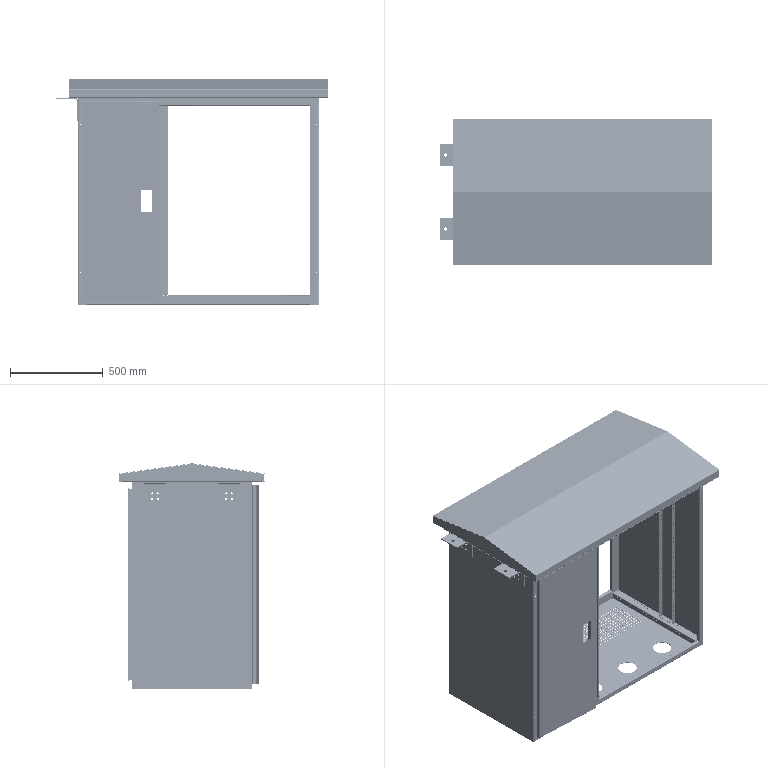Assembly | SolidWorks | mm | 23 component files | 23 solids | 4118 faces | box 1470 x 790 x 1217.97 mm | volume 9952438 mm3 | cylinder 2496 | plane 1582 | spline 40 | commonest cylinder face diameters 5 x1062 7 x724 5.4 x416 6 x80 3 x68 9 x40 13 x32 4 x20
Bill of materials:
BottomPlate4 | 1 |  | Rectangular sheet-metal tray-like panel: flat base with upturned walls along both long edges, each ending in a short outward flange, perforated by large round holes and arrays of short slots.
BottomPlateMiddleBeam | 1 |  | Long straight U-channel (open three-sided section, rounded bends) perforated with regularly spaced round holes on the web and both legs.
BottomSideBeam | 2 |  | Long straight channel with an asymmetric profile: web with one short leg and one long leg ending in an inward return lip; single rows of round holes on two faces.
BoxSidePlate01 | 2 |  | Flat rectangular sheet panel with formed flanges along two opposite edges, two clusters of four small holes near one end, and small holes in the flanges.
BoxUpperBeam2 | 1 |  | Long formed sheet-metal rail with a stepped Z/J-like profile (top flange, tall web, bottom flange, short upturned lip), with a row of oblong holes in the top flange and a rectangular notch in the lower flange.
BoxUpperBeam2Rear | 1 |  | Long formed sheet-metal rail with a stepped profile like the previous rail but mirrored, with four holes along one flange and a rectangular notch.
DoorPanel415 | 1 |  | Flat rectangular plate with a single off-center rectangular through-cutout.
LiftingBentPlate | 2 |  | Sheet-metal L-shaped angle bracket with a generous bend radius; one leg has one larger round hole, the other leg has a 2x2 pattern of four smaller round holes.
MiddleColumn3 | 2 |  | Long straight lipped C-channel with rounded corners and inward-turned lips, with no visible holes.
MountingColumn | 2 |  | Tall slender closed or folded rectangular-section post with a single row of small round holes along one narrow face and an end face with two oblong slots.
MountingColumnMiddle | 1 |  | Tall rectangular-section post, wider than the similar single-row post, with two rows of small round holes along one face and an end face with four oblong slots in a 2x2 pattern.
TopCover | 1 |  | Rectangular sheet-metal cover with a shallow peaked (gabled) top: two sloped panels meet at a central ridge, with short downturned side flanges ending in small inward lips.
TopCoverEndPlate | 2 |  | Thin flat sheet panel with a five-sided outline: a rectangle with a shallow triangular peak along one long edge. A narrow flange is bent at 90 degrees along the opposite straight long edge, with a small inside bend radius, so the cross-section is L-shaped.
TopCoverFrontAndRearFlange | 2 |  | Long, narrow sheet-metal strip with a Z-shaped (joggle) offset cross-section that forms two parallel flat flanges at different levels. The wider flange has one long row of many evenly spaced, identical narrow slots running along its length. The other flange is a little shorter, which leaves a step at each end, and has four small round or slightly oblong holes spaced along it.
TopCoverLeftAndRightFlange | 2 |  | Long sheet-metal strip with a Z-shaped (joggle) offset cross-section that forms two parallel flat flanges joined by a short perpendicular web with rounded bends. One flange has a single row of evenly spaced, identical narrow slots along its length. The other flange is plain and a little shorter, so the ends are offset or stepped.
Mates:
1. coincident | BottomPlate4-1 face at (-663.503, -344.148, 23.5) dir (0, -1, 0) | BoxSidePlate01-1 face at (538.497, -344.148, 1060) dir (0, -1, 0)
2. coincident | BottomPlate4-1 face at (-712.003, 322.852, -25) dir (0, 0, -1) | BoxSidePlate01-1 face at (583.997, -322.648, -25) dir (0, 0, -1)
3. distance | BottomPlate4-1 face at (584.997, 322.852, -25) dir (1, 0, 0) | BoxSidePlate01-1 face at (585.497, 324.352, -25) dir (-1, 0, 0)
4. coincident | BoxSidePlate01-1 face at (538.497, -344.148, 1060) dir (0, -1, 0) | BoxUpperBeam2-1 face at (-663.003, -344.148, 1050) dir (0, -1, 0)
5. coincident | BoxSidePlate01-1 face at (583.997, -324.148, 1100) dir (0, 0, 1) | BoxUpperBeam2-1 face at (-663.003, -300.648, 1100) dir (0, 0, 1)
6. coincident | BoxSidePlate01-1 face at (536.997, -324.148, -25) dir (-1, 0, 0) | BoxUpperBeam2-1 face at (536.997, -322.648, 1100) dir (1, 0, 0)
7. coincident | BoxUpperBeam2-1 face at (-663.003, -344.148, 1050) dir (0, -1, 0) | MiddleColumn3-1 face at (-288.003, -344.148, 25) dir (0, -1, 0)
8. coincident | BoxUpperBeam2-1 face at (-298.003, -324.148, 1050) dir (1, 0, 0) | MiddleColumn3-1 face at (-298.003, -344.148, 25) dir (-1, 0, 0)
9. coincident | BoxUpperBeam2-1 face at (-663.003, -324.148, 1050) dir (0, 0, -1) | MiddleColumn3-1 face at (-295.003, -342.648, 1050) dir (0, 0, 1)
10. coincident | BoxSidePlate01-1 face at (536.997, 324.352, -25) dir (0, 1, 0) | BoxUpperBeam2Rear-3 face at (536.997, 324.352, 1098.5) dir (0, 1, 0)
11. coincident | BoxSidePlate01-1 face at (585.497, -322.648, 1100) dir (0, 0, 1) | BoxUpperBeam2Rear-3 face at (536.997, 299.352, 1100) dir (0, 0, 1)
12. coincident | BoxSidePlate01-1 face at (536.997, 324.352, -25) dir (-1, 0, 0) | BoxUpperBeam2Rear-3 face at (536.997, 325.852, 1051.5) dir (1, 0, 0)
13. coincident | BottomPlate4-1 face at (-663.503, -344.148, 23.5) dir (0, -1, 0) | BoxSidePlate01-2 face at (-665.003, -344.148, 1060) dir (0, -1, 0)
14. coincident | BottomPlate4-1 face at (-712.003, 322.852, -25) dir (0, 0, -1) | BoxSidePlate01-2 face at (-712.003, -322.648, -25) dir (0, 0, -1)
15. coincident | BottomPlate4-1 face at (-712.003, 322.852, -15) dir (-1, 0, 0) | BoxSidePlate01-2 face at (-712.003, -325.648, -25) dir (1, 0, 0)
16. distance | BoxSidePlate01-2 face at (-712.003, -325.648, -25) dir (1, 0, 0) | BottomSideBeam-1 face at (-711.003, 321.852, 1.5) dir (-1, 0, 0)
17. coincident | BottomPlate4-1 face at (-712.003, 322.852, -23.5) dir (0, 0, 1) | BottomSideBeam-1 face at (-666.003, 321.852, -23.5) dir (0, 0, -1)
18. distance | BoxSidePlate01-2 face at (-663.503, -325.648, -25) dir (0, -1, 0) | BottomSideBeam-1 face at (-670.003, -323.148, 9.5) dir (0, -1, 0)
19. coincident | BottomPlate4-1 face at (-712.003, 322.852, -23.5) dir (0, 0, 1) | BottomPlateMiddleBeam-1 face at (-288.503, -323.148, -23.5) dir (0, 0, -1)
20. distance | BottomPlate4-1 face at (-663.503, -325.648, 25) dir (0, -1, 0) | BottomPlateMiddleBeam-1 face at (-239.503, -323.148, 7.5) dir (0, -1, 0)
21. distance | BottomPlateMiddleBeam-1 face at (-290.503, -323.148, -23.5) dir (-1, 0, 0) | MiddleColumn3-1 face at (-298.003, -344.148, 25) dir (-1, 0, 0)
22. coincident | BottomPlate4-1 face at (-712.003, 322.852, -23.5) dir (0, 0, 1) | BottomSideBeam-2 face at (539.497, -323.148, -23.5) dir (0, 0, -1)
23. distance | BoxSidePlate01-1 face at (585.497, 324.352, -25) dir (-1, 0, 0) | BottomSideBeam-2 face at (584.497, -323.148, 1.5) dir (1, 0, 0)
24. distance | BoxSidePlate01-1 face at (536.997, 324.352, -25) dir (0, 1, 0) | BottomSideBeam-2 face at (543.497, 321.852, 9.5) dir (0, 1, 0)
25. distance | MountingColumn-1 face at (584.497, -113.148, 1061.5) dir (0, -1, 0) | BoxSidePlate01-1 face at (586.997, -325.648, -25) dir (0, -1, 0)
26. coincident | BottomSideBeam-2 face at (584.497, -323.148, 11.5) dir (0, 0, 1) | MountingColumn-1 face at (559.497, -17.148, 11.5) dir (0, 0, -1)
27. distance | MountingColumn-1 face at (584.497, -13.148, 1061.5) dir (1, 0, 0) | BoxSidePlate01-1 face at (585.497, 324.352, -25) dir (-1, 0, 0)
28. coincident | BottomPlateMiddleBeam-1 face at (-235.503, -323.148, 11.5) dir (1, 0, 0) | MountingColumnMiddle-1 face at (-235.503, -13.148, 961.5) dir (1, 0, 0)
29. distance | MountingColumnMiddle-1 face at (-235.503, -113.148, 961.5) dir (0, -1, 0) | MiddleColumn3-1 face at (-298.003, -325.648, 25) dir (0, -1, 0)
30. coincident | BottomPlateMiddleBeam-1 face at (-290.503, -323.148, 11.5) dir (0, 0, 1) | MountingColumnMiddle-1 face at (-290.503, -17.148, 11.5) dir (0, 0, -1)
31. distance | BoxSidePlate01-2 face at (-663.503, -325.648, -25) dir (0, -1, 0) | MountingColumn-2 face at (-686.003, -113.148, 1061.5) dir (0, -1, 0)
32. distance | BoxSidePlate01-2 face at (-712.003, -325.648, -25) dir (1, 0, 0) | MountingColumn-2 face at (-711.003, -113.148, 1061.5) dir (-1, 0, 0)
33. coincident | BottomSideBeam-1 face at (-711.003, 321.852, 11.5) dir (0, 0, 1) | MountingColumn-2 face at (-686.003, -109.148, 11.5) dir (0, 0, -1)
34. distance | BoxSidePlate01-2 face at (-713.503, -325.648, -25) dir (-1, 0, 0) | TopCoverAssembly-1/TopCoverEndPlate-2 face at (-763.503, 391.852, 1244.7) dir (-1, 0, 0)
35. distance | BoxSidePlate01-2 face at (-713.503, 324.352, -25) dir (0, 1, 0) | TopCoverAssembly-1/TopCover-1 face at (636.497, 394.352, 1093) dir (0, 1, 0)
36. coincident | BoxUpperBeam2Rear-3 face at (536.997, 299.352, 1100) dir (0, 0, 1) | TopCoverAssembly-1/TopCoverFrontAndRearFlange-1 face at (-761.003, 328.352, 1100) dir (0, 0, -1)
37. coincident | BoxSidePlate01-2 face at (-713.503, -325.648, -25) dir (-1, 0, 0) | LiftingBentPlate-1 face at (-713.503, 139.352, 1090) dir (1, 0, 0)
38. concentric | BoxSidePlate01-2 edge at (-713.503, 214.352, 1030) dir (-1, 0, 0) r 6.5 | LiftingBentPlate-1 edge at (-719.503, 214.352, 1030) dir (-1, 0, 0) r 5.5
39. concentric | BoxSidePlate01-2 edge at (-712.003, 184.352, 1030) dir (1, 0, 0) r 6.5 | LiftingBentPlate-1 edge at (-719.503, 184.352, 1030) dir (-1, 0, 0) r 5.5
40. parallel | BoxSidePlate01-2 face at (-710.503, 322.852, -25) dir (0, 0, -1) | DoorPanel415-1 face at (-278.243, -363.153, 0) dir (0, 0, -1)
41. coincident | TopCover-1 face at (43.278, -378.459, 700) dir (0, 0, 1) | TopCoverEndPlate-1 face at (-106.922, -377.959, 700) dir (0, 0, 1)
42. coincident | TopCover-1 face at (44.778, -381.459, 700) dir (1, 0, 0) | TopCoverEndPlate-1 face at (44.778, -364.959, 698.5) dir (1, 0, 0)
43. distance | TopCover-1 face at (44.778, 407.041, 700) dir (0, -1, 0) | TopCoverEndPlate-1 face at (42.778, 406.041, 698.5) dir (0, 1, 0)
44. coincident | TopCoverEndPlate-1 face at (44.778, -364.959, 698.5) dir (1, 0, 0) | TopCoverLeftAndRightFlange-1 face at (44.778, 339.541, 700) dir (-1, 0, 0)
45. distance | TopCover-1 face at (44.778, 408.541, 700) dir (0, 1, 0) | TopCoverLeftAndRightFlange-1 face at (43.278, 339.541, 655.5) dir (0, 1, 0)
46. coincident | TopCoverEndPlate-1 face at (-106.922, -377.959, 700) dir (0, 0, 1) | TopCoverLeftAndRightFlange-1 face at (46.278, 339.541, 700) dir (0, 0, 1)
47. coincident | TopCover-1 face at (44.778, 408.541, 700) dir (1, 0, 0) | TopCoverFrontAndRearFlange-1 face at (44.778, 408.541, -697.5) dir (-1, 0, 0)
48. coincident | TopCover-1 face at (44.778, 408.541, 700) dir (0, 1, 0) | TopCoverFrontAndRearFlange-1 face at (46.278, 408.541, -697.5) dir (0, 1, 0)
49. distance | TopCover-1 face at (0.9031, 405.748, 700) dir (0, 0, 1) | TopCoverFrontAndRearFlange-1 face at (39.278, 341.041, 697.5) dir (0, 0, 1)